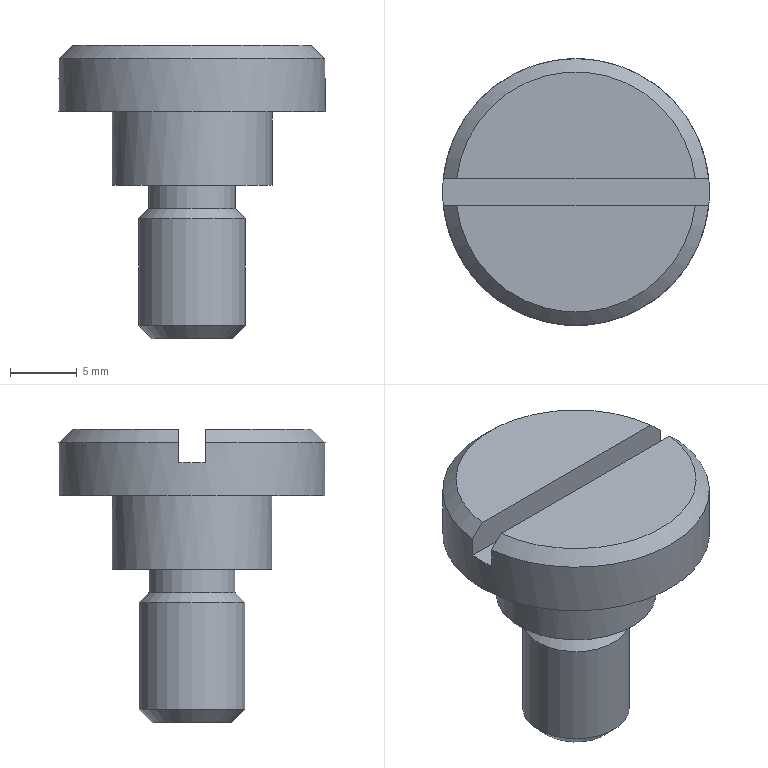Component | NX | BORING_SLEEVE_SCREW | 1 solid | 16 faces | volume 2595 mm3 | plane 8 | cylinder 4 | cone 4 | commonest cylinder face diameters 8 x1 6.5 x1 12 x1 20 x1